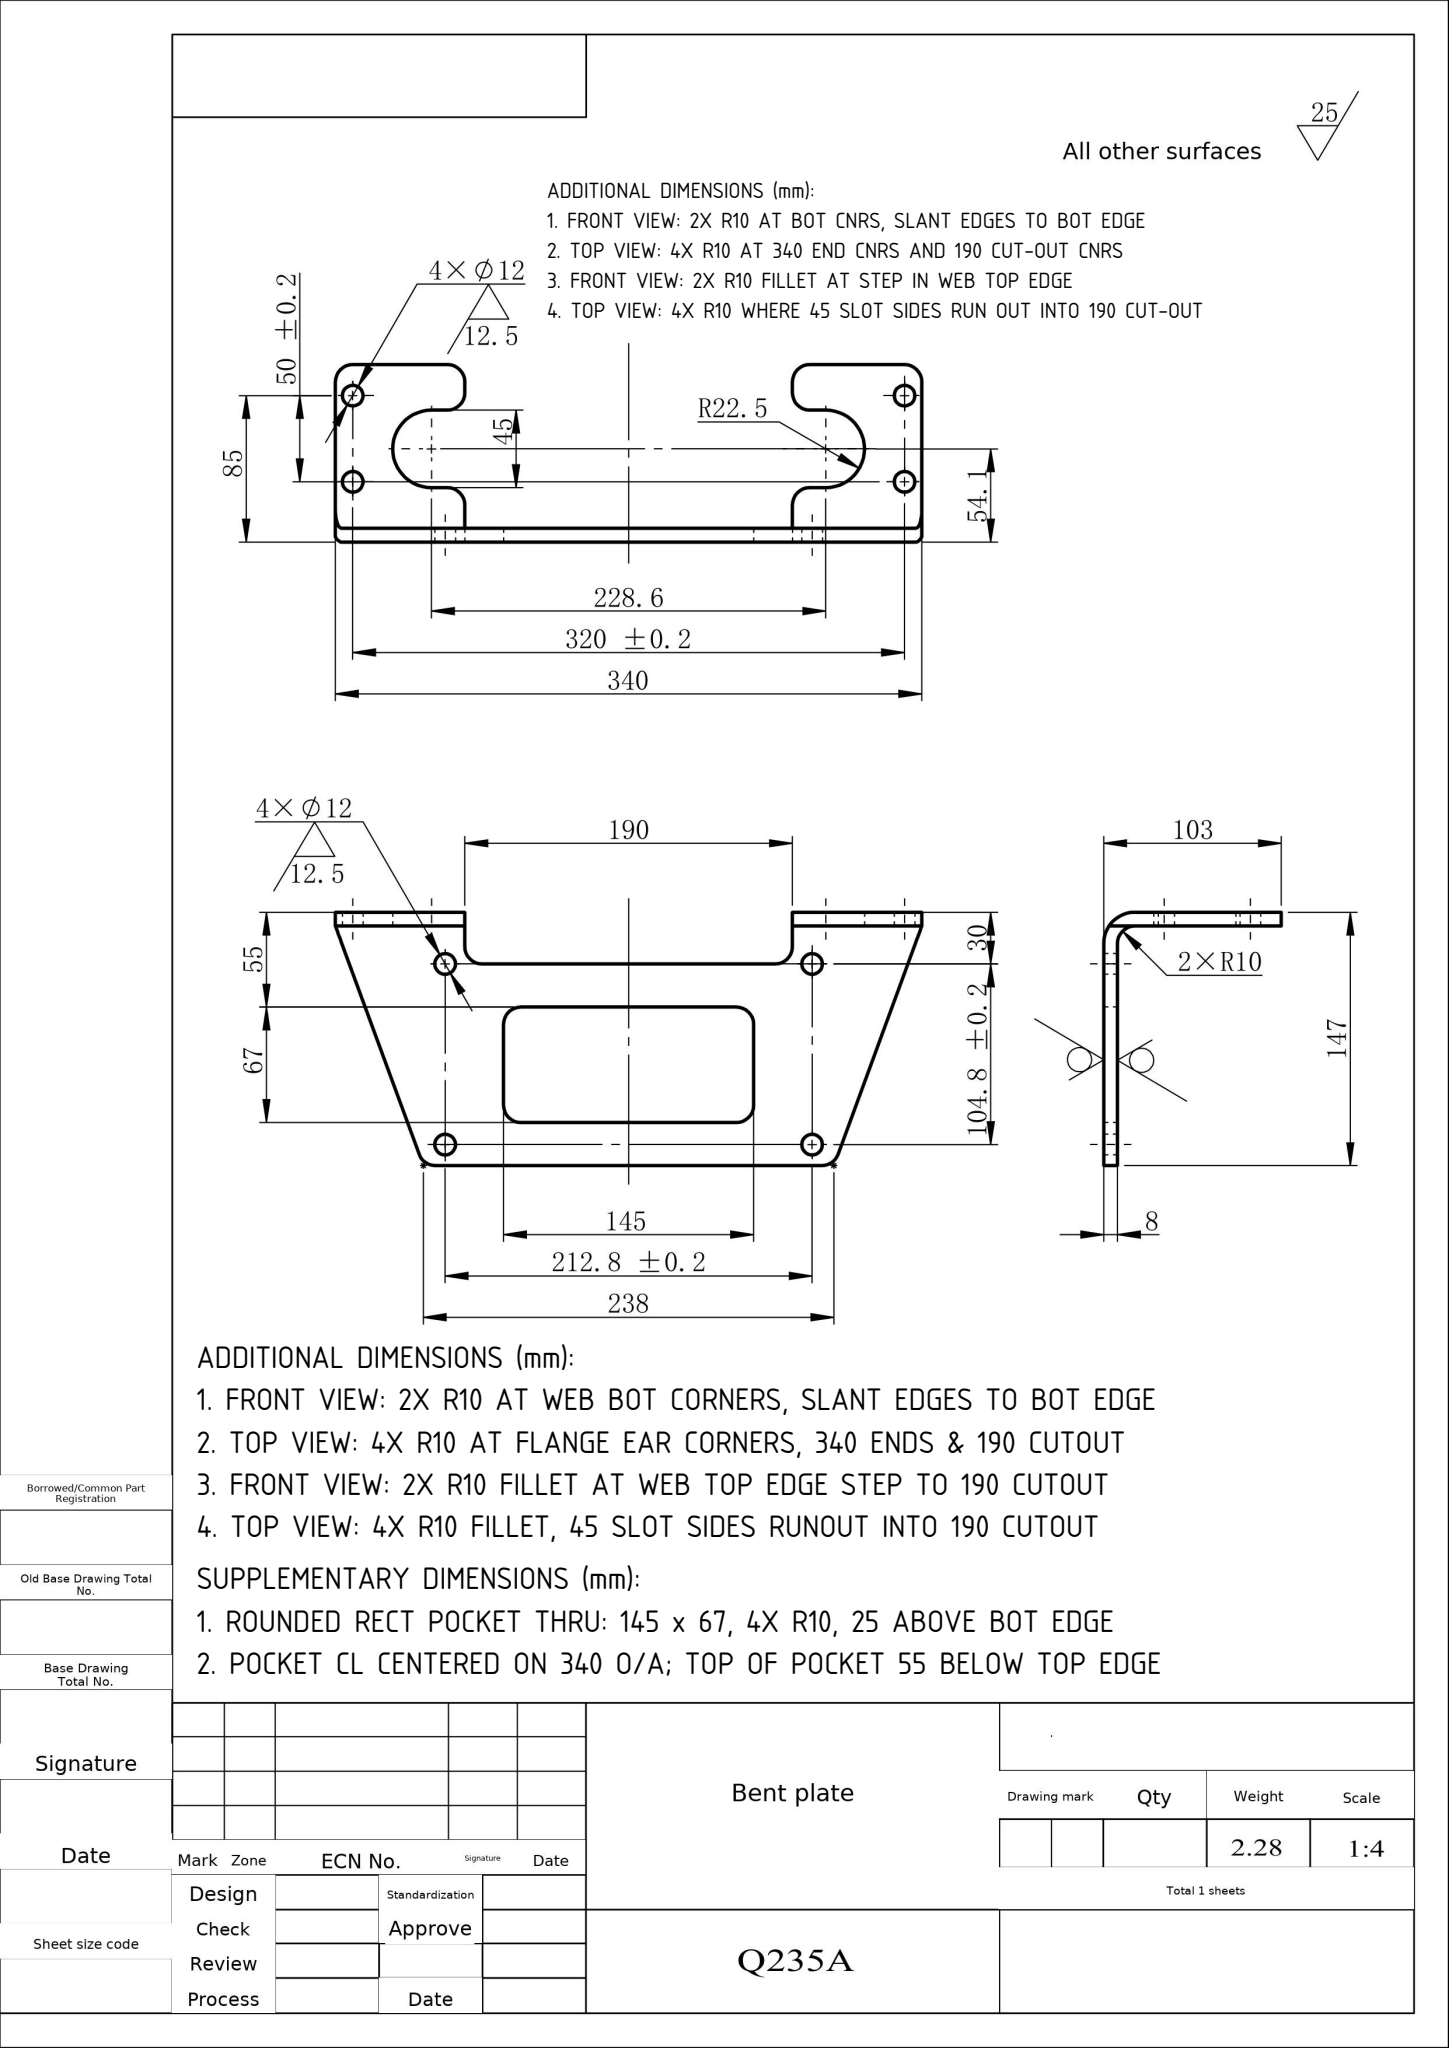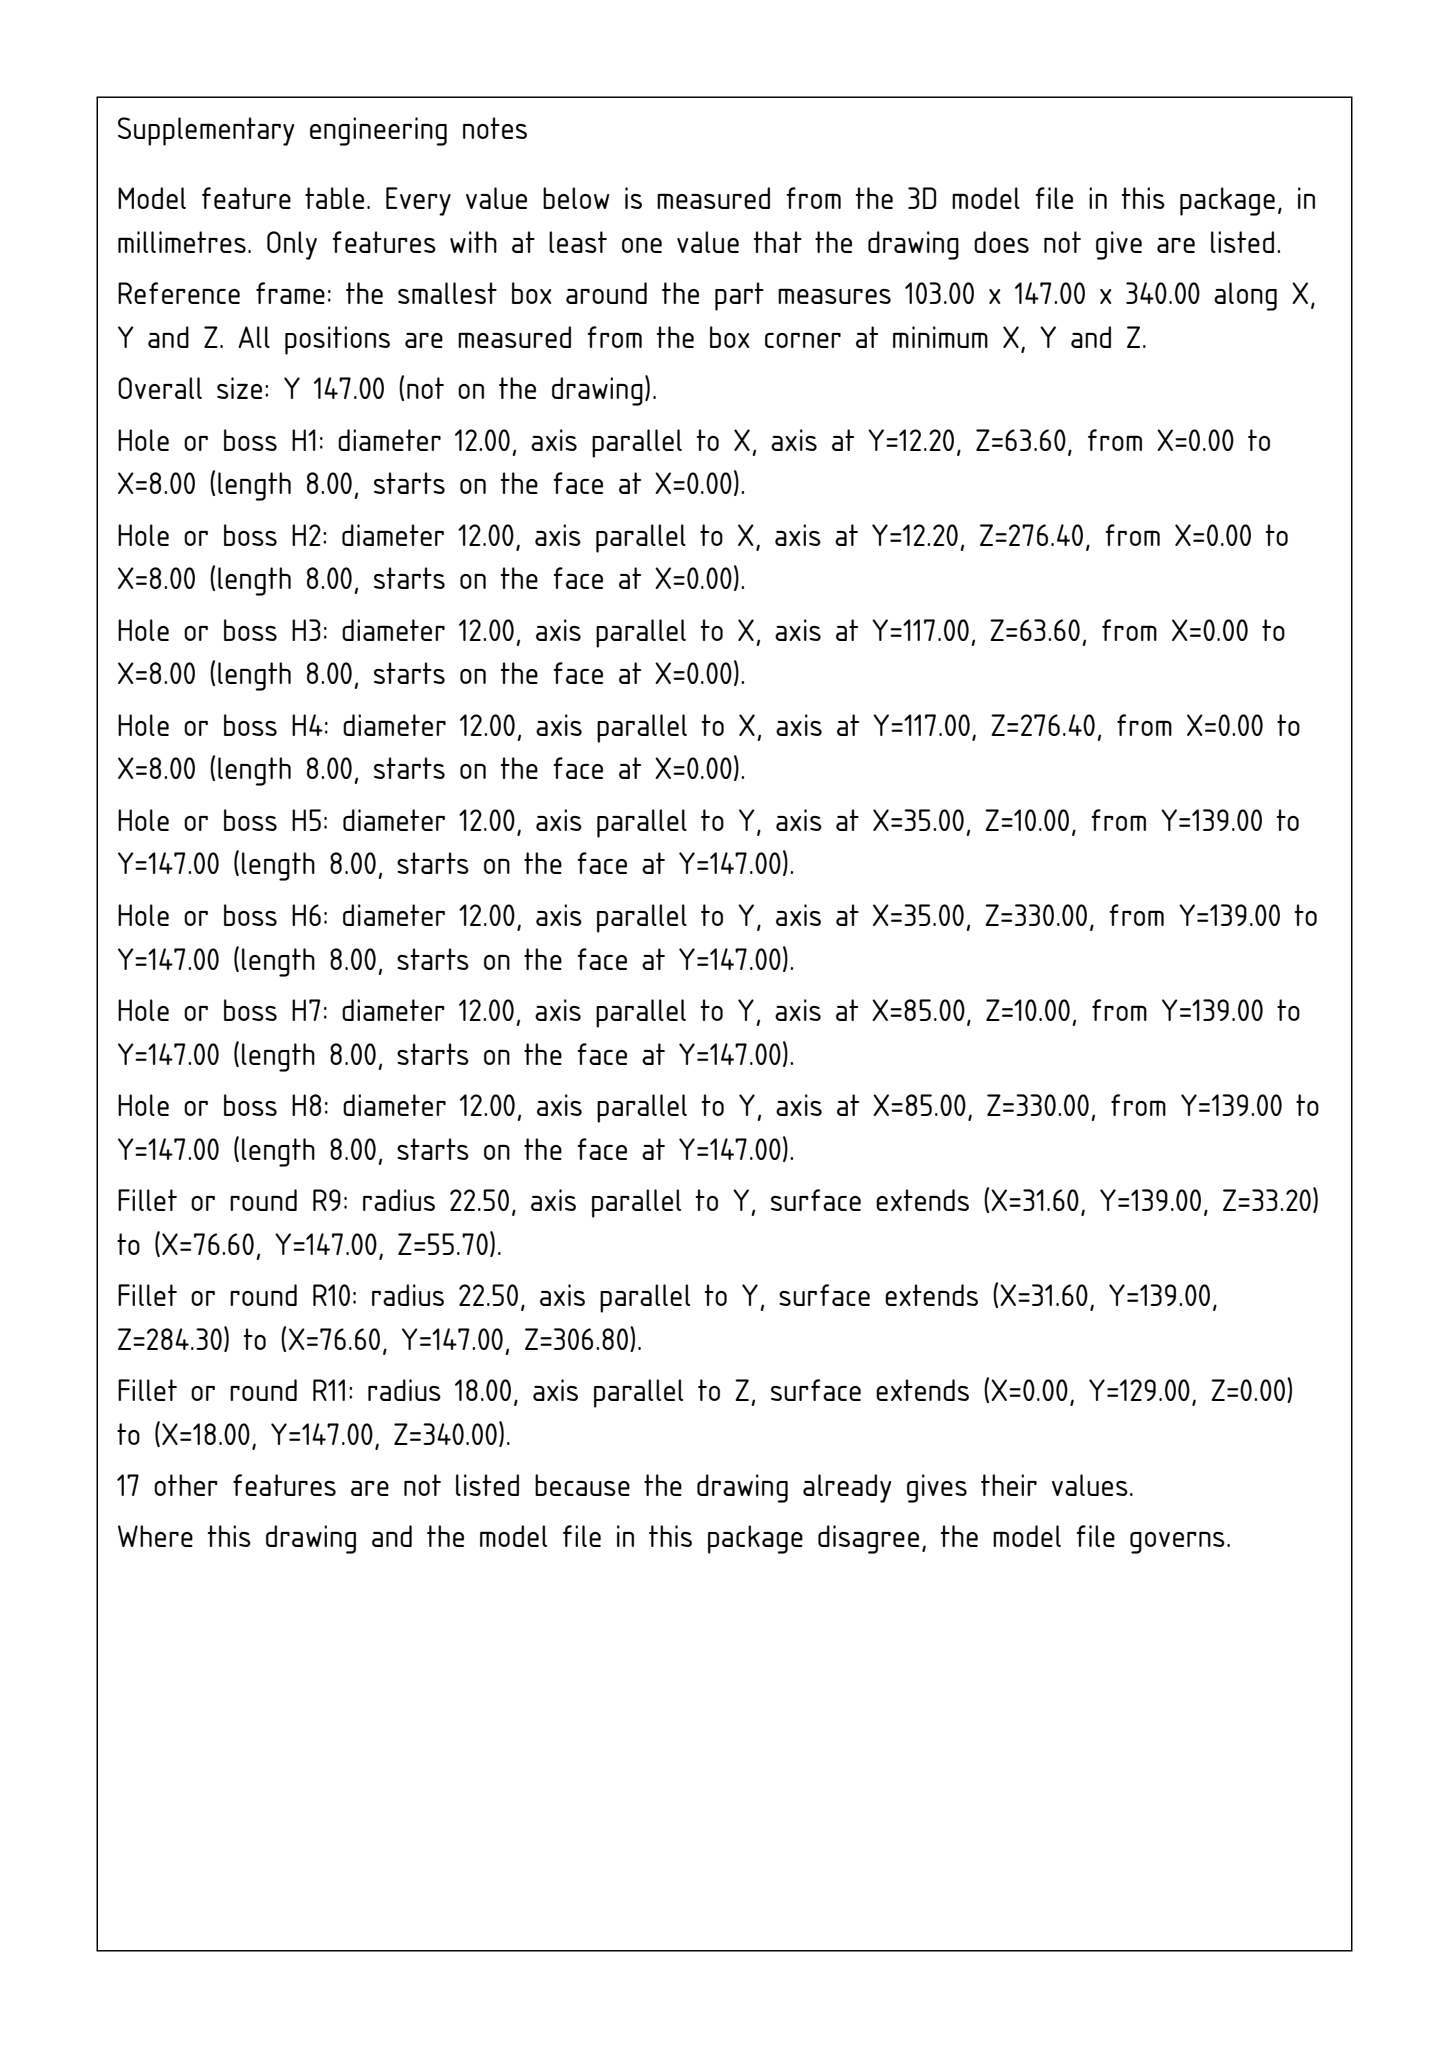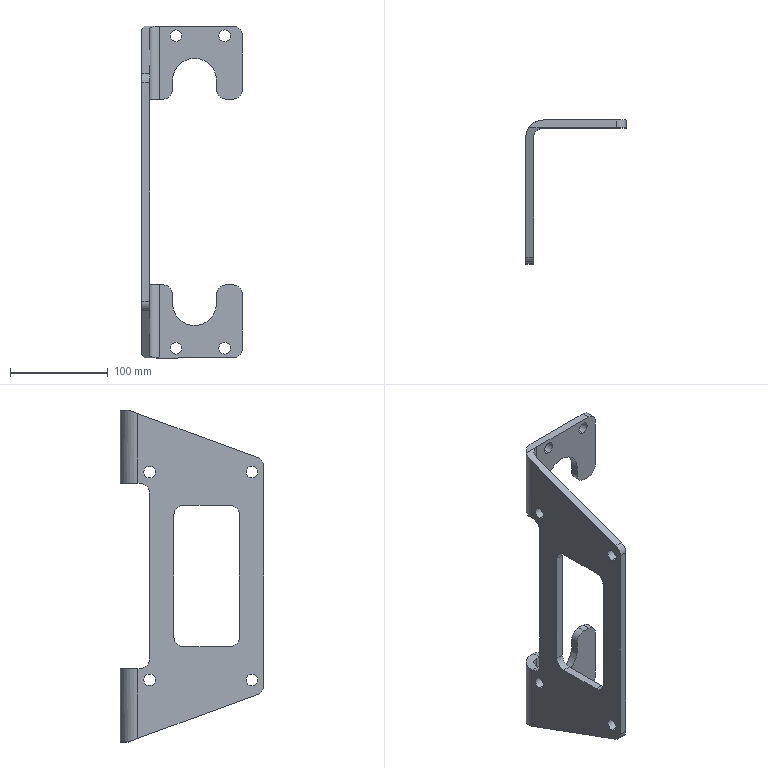Part | SolidWorks | mm | 1 solid | 65 faces | box 103 x 147 x 340 mm | volume 292237 mm3 | cylinder 39 | plane 26 | commonest cylinder face diameters 20 x18 12 x16 45 x3 36 x2
build123d program:
from build123d import *

# Parameters (mm, degrees)
SKETCH6_W                  = 285
SKETCH6_H                  = 147
BOSS_EXTRUDE1_DEPTH        = 8
SKETCH9_R                  = 6
CUT_EXTRUDE2_DEPTH         = 161.538
SKETCH11_W                 = 23.5
SKETCH11_H                 = 17
CUT_EXTRUDE3_DEPTH         = 161.538
SKETCH12_W                 = 340
SKETCH12_H                 = 8
BOSS_EXTRUDE3_DEPTH        = 95
SKETCH13_W                 = 180
SKETCH13_H                 = 190
CUT_EXTRUDE4_DEPTH         = 30
F_12_0_12_DIAMETER_HOLE1_D = 12
SKETCH35_W                 = 12
SKETCH35_H                 = 27.5
CUT_EXTRUDE5_DEPTH         = 10
SKETCH36_W                 = 145
SKETCH36_H                 = 67
CUT_EXTRUDE6_DEPTH         = 10
CUT_EXTRUDE7_DEPTH         = 248.221
BOSS_EXTRUDE4_DEPTH        = 27.5
BOSS_EXTRUDE6_DEPTH        = 8
CUT_EXTRUDE8_DEPTH         = 209.152
FILLET1_R                  = 10
FILLET2_R                  = 18
FILLET3_R                  = 10
FILLET4_R                  = 10


with BuildPart() as part:
    # Sketch6 → Boss-Extrude1 (new body)
    with BuildSketch(Plane(origin=(0, 0, 0), x_dir=(0, 0, -1), z_dir=(1, 0, 0))):
        Rectangle(SKETCH6_W, SKETCH6_H)
    extrude(amount=BOSS_EXTRUDE1_DEPTH)

    # Sketch9 → Cut-Extrude2 (cut, through all)
    with BuildSketch(Plane.ZY):
        with Locations((-106.4, 43.5)):
            Circle(SKETCH9_R)
        with Locations((-106.4, -61.3)):
            Circle(SKETCH9_R)
        with Locations(Location((106.4, -61.3, 0), (0, 0, 180))):
            Circle(SKETCH9_R)
        with Locations(Location((106.4, 43.5, 0), (0, 0, 180))):
            Circle(SKETCH9_R)
    extrude(amount=-CUT_EXTRUDE2_DEPTH, mode=Mode.SUBTRACT)

    # Sketch11 → Cut-Extrude3 (cut, through all)
    with BuildSketch(Plane(origin=(8, 0, 0), x_dir=(0, 0, -1), z_dir=(1, 0, 0))):
        with Locations((-130.75, -65)):
            Rectangle(SKETCH11_W, SKETCH11_H)
        with Locations((130.75, -65)):
            Rectangle(SKETCH11_W, SKETCH11_H)
    extrude(amount=-CUT_EXTRUDE3_DEPTH, mode=Mode.SUBTRACT)

    # Sketch12 → Boss-Extrude3 (add)
    with BuildSketch(Plane(origin=(8, 0, 0), x_dir=(0, 0, -1), z_dir=(1, 0, 0))):
        with Locations((0, 69.5)):
            Rectangle(SKETCH12_W, SKETCH12_H)
    extrude(amount=BOSS_EXTRUDE3_DEPTH)

    # Sketch13 → Cut-Extrude4 (cut)
    with BuildSketch(Plane(origin=(0, 73.5, 0), x_dir=(1, 0, 0), z_dir=(0, 1, 0))):
        with Locations((82, 0)):
            Rectangle(SKETCH13_W, SKETCH13_H)
    extrude(amount=-CUT_EXTRUDE4_DEPTH, mode=Mode.SUBTRACT)

    # 12.0 _12_ Diameter Hole1 (through all)
    with Locations(Plane(origin=(0, 73.5, 0), x_dir=(1, 0, 0), z_dir=(0, 1, 0))):
        with Locations((85, 160), (35, 160), (35, -160), (85, -160)):
            Hole(F_12_0_12_DIAMETER_HOLE1_D / 2)

    # Sketch35 → Cut-Extrude5 (cut)
    with BuildSketch(Plane(origin=(0, 73.5, 0), x_dir=(1, 0, 0), z_dir=(0, 1, 0))):
        with Locations((14, 156.25)):
            Rectangle(SKETCH35_W, SKETCH35_H)
        with Locations((14, -156.25)):
            Rectangle(SKETCH35_W, SKETCH35_H)
    extrude(amount=-CUT_EXTRUDE5_DEPTH, mode=Mode.SUBTRACT)

    # Sketch36 → Cut-Extrude6 (cut)
    with BuildSketch(Plane.ZY):
        with Locations((0, -15)):
            Rectangle(SKETCH36_W, SKETCH36_H)
    extrude(amount=-CUT_EXTRUDE6_DEPTH, mode=Mode.SUBTRACT)

    # Sketch37 → Cut-Extrude7 (cut, through all)
    with BuildSketch(Plane(origin=(0, 73.5, 0), x_dir=(1, 0, 0), z_dir=(0, 1, 0))):
        with BuildLine():
            Line((31.6, 95), (76.6, 95))
            Line((76.6, 95), (76.6, 114.3))
            ThreePointArc((76.6, 114.3), (54.1, 136.8), (31.6, 114.3))
            Line((31.6, 114.3), (31.6, 95))
        make_face()
        with BuildLine():
            Line((76.6, -114.3), (76.6, -95))
            Line((76.6, -95), (31.6, -95))
            Line((31.6, -95), (31.6, -114.3))
            ThreePointArc((31.6, -114.3), (54.1, -136.8), (76.6, -114.3))
        make_face()
    extrude(amount=-CUT_EXTRUDE7_DEPTH, mode=Mode.SUBTRACT)

    # Sketch38 → Boss-Extrude4 (add)
    with BuildSketch(Plane.XY.offset(142.5)):
        Polygon((20, 73.5), (0, 73.5), (0, -56.5), (8, -56.5), (8, 65.5), (20, 65.5), align=None)
    boss_extrude4 = extrude(amount=BOSS_EXTRUDE4_DEPTH)

    # Sketch40 → Boss-Extrude6 (add)
    with BuildSketch(Plane(origin=(8, 0, 0), x_dir=(0, 0, -1), z_dir=(1, 0, 0))):
        Polygon((-119, -56.5), (-170, -56.5), (-119, -73.5), align=None)
    boss_extrude6 = extrude(amount=-BOSS_EXTRUDE6_DEPTH)

    # Sketch41 → Cut-Extrude8 (cut, through all)
    with BuildSketch(Plane(origin=(8, 0, 0), x_dir=(0, 0, -1), z_dir=(1, 0, 0))):
        Polygon((-170, 65.5), (-119, -73.5), (-170, -73.5), align=None)
    cut_extrude8 = extrude(amount=-CUT_EXTRUDE8_DEPTH, mode=Mode.SUBTRACT)

    # Mirror1: Boss-Extrude4, Boss-Extrude6, Cut-Extrude8 across plane
    add(boss_extrude4.mirror(Plane.XY))
    add(boss_extrude6.mirror(Plane.XY))
    add(cut_extrude8.mirror(Plane.XY), mode=Mode.SUBTRACT)

    # Fillet1
    fillet1_edges = [part.edges().sort_by_distance(p)[0] for p in [
        (8, 65.5, 132.5),
        (8, 65.5, -132.5),
    ]]
    fillet(fillet1_edges, radius=FILLET1_R)

    # Fillet2
    fillet2_edges = [part.edges().sort_by_distance(p)[0] for p in [
        (0, 73.5, -132.5),
        (0, 73.5, 132.5),
    ]]
    fillet(fillet2_edges, radius=FILLET2_R)

    # Fillet3
    fillet3_edges = [part.edges().sort_by_distance(p)[0] for p in [
        (4, -48.5, -72.5),
        (4, 18.5, -72.5),
        (4, 18.5, 72.5),
        (4, -48.5, 72.5),
    ]]
    fillet(fillet3_edges, radius=FILLET3_R)

    # Fillet4
    fillet4_edges = [part.edges().sort_by_distance(p)[0] for p in [
        (31.6, 69.5, -95),
        (76.6, 69.5, -95),
        (76.6, 69.5, 95),
        (31.6, 69.5, 95),
        (4, -73.5, 119),
        (4, -73.5, -119),
        (103, 69.5, 170),
        (103, 69.5, -170),
        (103, 69.5, 95),
        (103, 69.5, -95),
        (4, 43.5, -95),
        (4, 43.5, 95),
    ]]
    fillet(fillet4_edges, radius=FILLET4_R)


solid = part.part